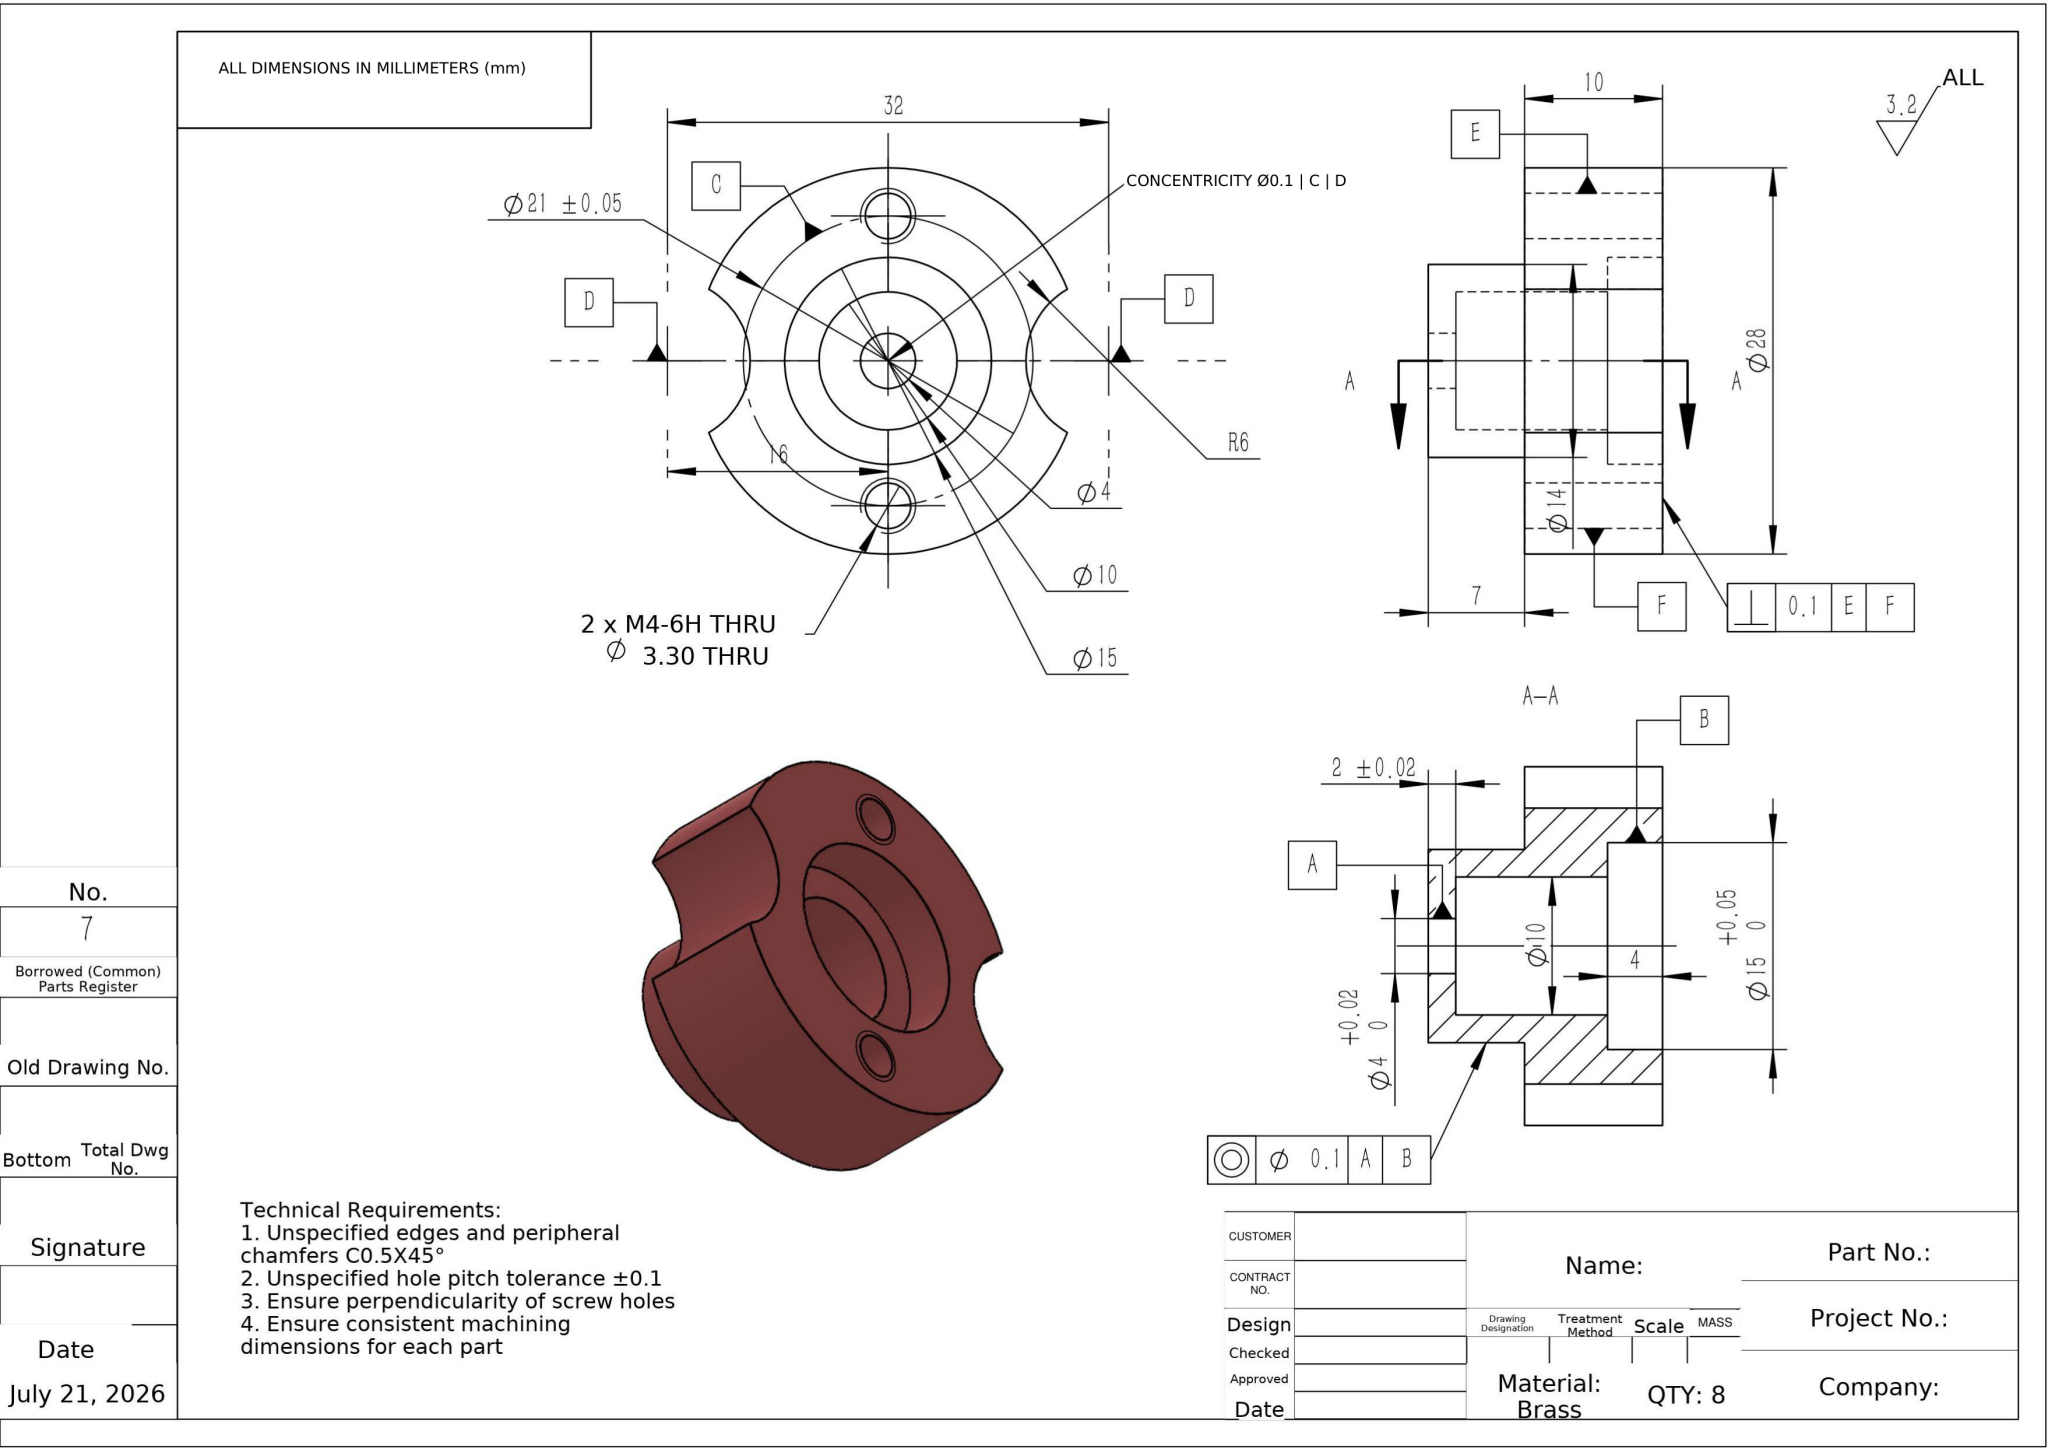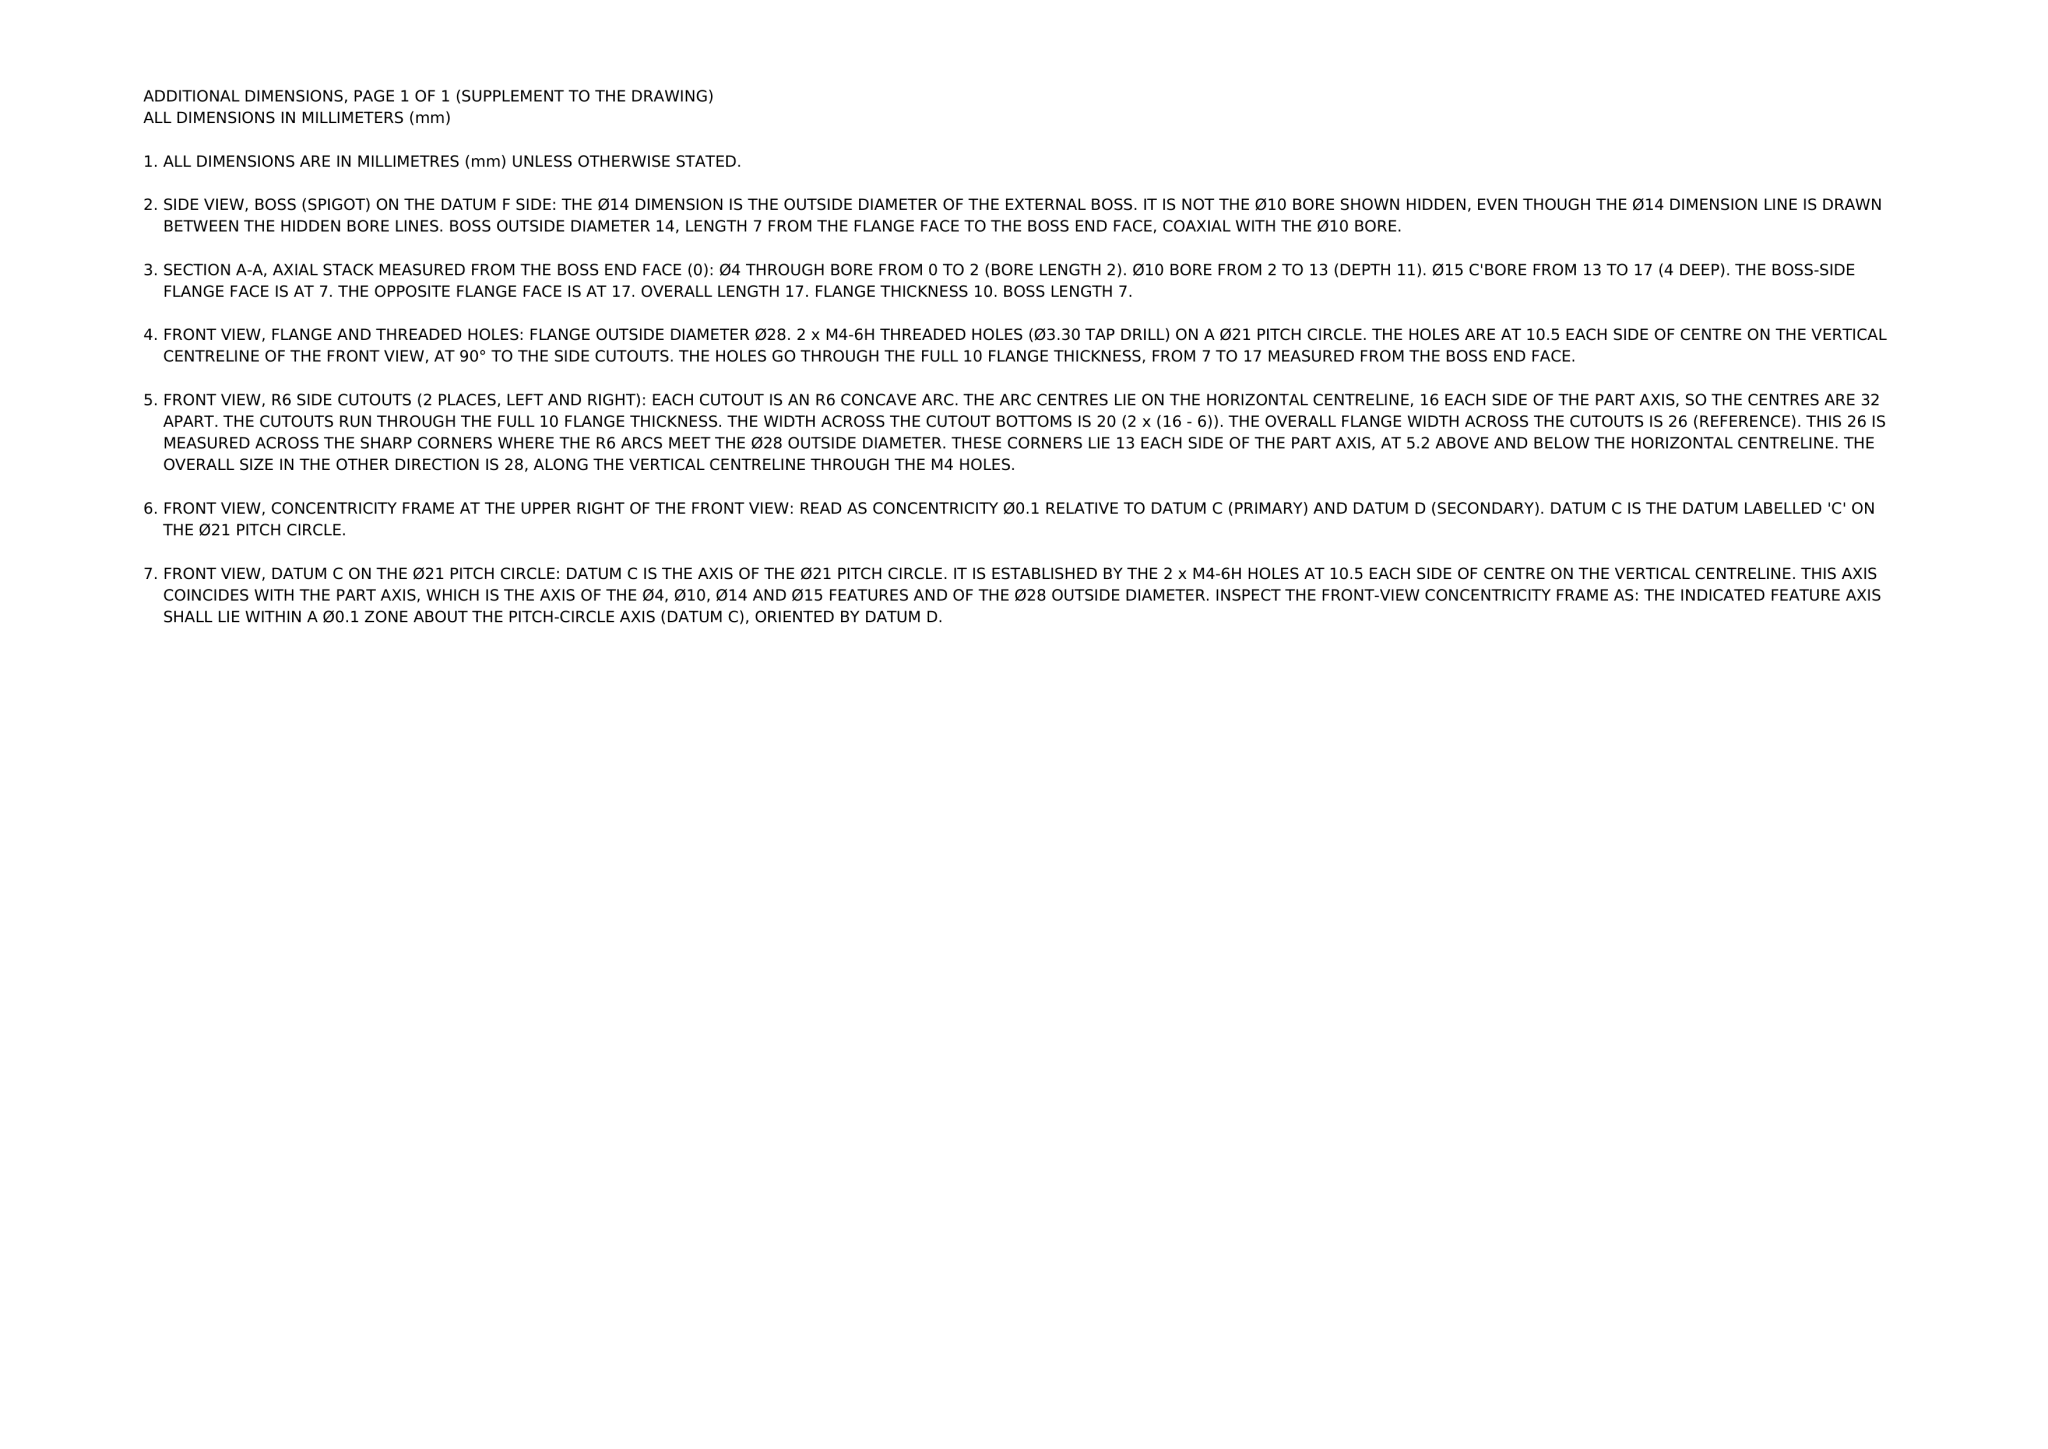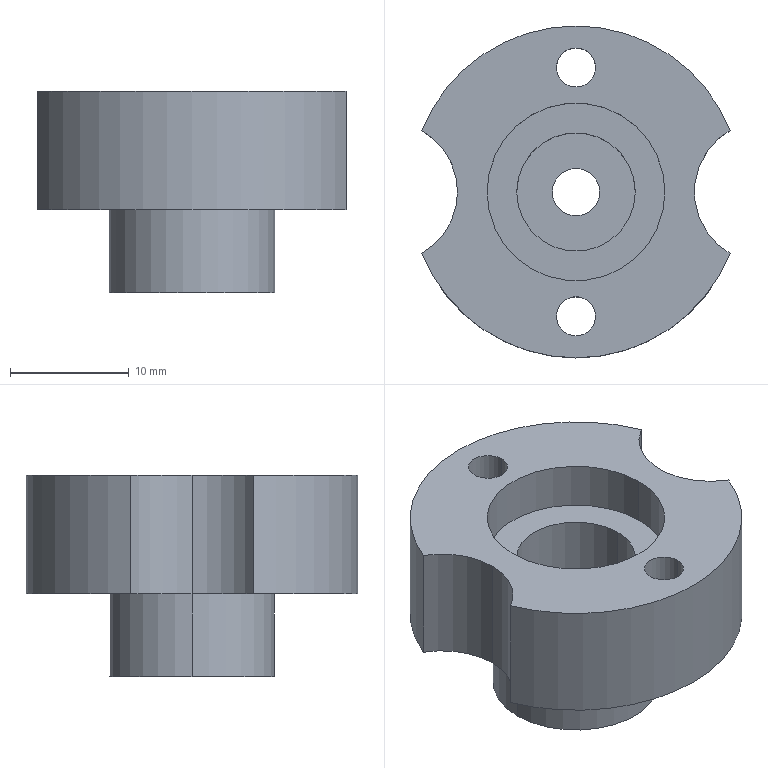Part | NX | mm | 1 solid | 22 faces | box 26 x 28 x 17 mm | volume 4886 mm3 | cylinder 17 | plane 5 | commonest cylinder face diameters 3.3 x4 12 x3 14 x2 4 x2 10 x2 15 x2 28 x2
STEP:
#1=CARTESIAN_POINT('',(1.65,10.5,7.));
#2=VERTEX_POINT('',#1);
#3=CARTESIAN_POINT('',(-1.65,10.5,7.));
#4=VERTEX_POINT('',#3);
#5=CARTESIAN_POINT('',(0.,10.5,7.));
#6=DIRECTION('',(0.,0.,-1.));
#7=DIRECTION('',(-1.,0.,0.));
#8=AXIS2_PLACEMENT_3D('',#5,#6,#7);
#9=CIRCLE('',#8,1.65);
#10=EDGE_CURVE('',#2,#4,#9,.T.);
#11=ORIENTED_EDGE('',*,*,#10,.T.);
#12=CARTESIAN_POINT('',(-1.65,10.5,17.));
#13=VERTEX_POINT('',#12);
#14=CARTESIAN_POINT('',(-1.65,10.5,17.));
#15=DIRECTION('',(0.,0.,1.));
#16=VECTOR('',#15,1000.);
#17=LINE('',#14,#16);
#18=EDGE_CURVE('',#4,#13,#17,.T.);
#19=ORIENTED_EDGE('',*,*,#18,.T.);
#20=CARTESIAN_POINT('',(1.65,10.5,17.));
#21=VERTEX_POINT('',#20);
#22=CARTESIAN_POINT('',(0.,10.5,17.));
#23=DIRECTION('',(0.,0.,1.));
#24=DIRECTION('',(1.,0.,0.));
#25=AXIS2_PLACEMENT_3D('',#22,#23,#24);
#26=CIRCLE('',#25,1.65);
#27=EDGE_CURVE('',#13,#21,#26,.T.);
#28=ORIENTED_EDGE('',*,*,#27,.T.);
#29=CARTESIAN_POINT('',(1.65,10.5,17.));
#30=DIRECTION('',(0.,0.,1.));
#31=VECTOR('',#30,1000.);
#32=LINE('',#29,#31);
#33=EDGE_CURVE('',#2,#21,#32,.T.);
#34=ORIENTED_EDGE('',*,*,#33,.F.);
#35=EDGE_LOOP('',(#11,#19,#28,#34));
#36=FACE_OUTER_BOUND('',#35,.T.);
#37=CARTESIAN_POINT('',(0.,10.5,17.));
#38=DIRECTION('',(0.,0.,1.));
#39=DIRECTION('',(1.,0.,0.));
#40=AXIS2_PLACEMENT_3D('',#37,#38,#39);
#41=CYLINDRICAL_SURFACE('',#40,1.65);
#42=ADVANCED_FACE('',(#36),#41,.F.);
#43=CARTESIAN_POINT('',(1.65,-10.5,7.));
#44=VERTEX_POINT('',#43);
#45=CARTESIAN_POINT('',(-1.65,-10.5,7.));
#46=VERTEX_POINT('',#45);
#47=CARTESIAN_POINT('',(0.,-10.5,7.));
#48=DIRECTION('',(0.,0.,-1.));
#49=DIRECTION('',(-1.,0.,0.));
#50=AXIS2_PLACEMENT_3D('',#47,#48,#49);
#51=CIRCLE('',#50,1.65);
#52=EDGE_CURVE('',#44,#46,#51,.T.);
#53=ORIENTED_EDGE('',*,*,#52,.T.);
#54=CARTESIAN_POINT('',(-1.65,-10.5,17.));
#55=VERTEX_POINT('',#54);
#56=CARTESIAN_POINT('',(-1.65,-10.5,17.));
#57=DIRECTION('',(0.,0.,1.));
#58=VECTOR('',#57,1000.);
#59=LINE('',#56,#58);
#60=EDGE_CURVE('',#46,#55,#59,.T.);
#61=ORIENTED_EDGE('',*,*,#60,.T.);
#62=CARTESIAN_POINT('',(1.65,-10.5,17.));
#63=VERTEX_POINT('',#62);
#64=CARTESIAN_POINT('',(0.,-10.5,17.));
#65=DIRECTION('',(0.,0.,1.));
#66=DIRECTION('',(1.,0.,0.));
#67=AXIS2_PLACEMENT_3D('',#64,#65,#66);
#68=CIRCLE('',#67,1.65);
#69=EDGE_CURVE('',#55,#63,#68,.T.);
#70=ORIENTED_EDGE('',*,*,#69,.T.);
#71=CARTESIAN_POINT('',(1.65,-10.5,17.));
#72=DIRECTION('',(0.,0.,1.));
#73=VECTOR('',#72,1000.);
#74=LINE('',#71,#73);
#75=EDGE_CURVE('',#44,#63,#74,.T.);
#76=ORIENTED_EDGE('',*,*,#75,.F.);
#77=EDGE_LOOP('',(#53,#61,#70,#76));
#78=FACE_OUTER_BOUND('',#77,.T.);
#79=CARTESIAN_POINT('',(0.,-10.5,17.));
#80=DIRECTION('',(0.,0.,1.));
#81=DIRECTION('',(1.,0.,0.));
#82=AXIS2_PLACEMENT_3D('',#79,#80,#81);
#83=CYLINDRICAL_SURFACE('',#82,1.65);
#84=ADVANCED_FACE('',(#78),#83,.F.);
#85=CARTESIAN_POINT('',(-7.,0.,7.));
#86=VERTEX_POINT('',#85);
#87=CARTESIAN_POINT('',(7.,0.,7.));
#88=VERTEX_POINT('',#87);
#89=CARTESIAN_POINT('',(0.,0.,7.));
#90=DIRECTION('',(0.,0.,-1.));
#91=DIRECTION('',(-1.,0.,0.));
#92=AXIS2_PLACEMENT_3D('',#89,#90,#91);
#93=CIRCLE('',#92,7.);
#94=EDGE_CURVE('',#86,#88,#93,.T.);
#95=ORIENTED_EDGE('',*,*,#94,.T.);
#96=CARTESIAN_POINT('',(7.,0.,0.));
#97=VERTEX_POINT('',#96);
#98=CARTESIAN_POINT('',(7.,0.,7.));
#99=DIRECTION('',(0.,0.,-1.));
#100=VECTOR('',#99,1000.);
#101=LINE('',#98,#100);
#102=EDGE_CURVE('',#88,#97,#101,.T.);
#103=ORIENTED_EDGE('',*,*,#102,.T.);
#104=CARTESIAN_POINT('',(-7.,0.,0.));
#105=VERTEX_POINT('',#104);
#106=CARTESIAN_POINT('',(0.,0.,0.));
#107=DIRECTION('',(0.,0.,-1.));
#108=DIRECTION('',(-1.,0.,0.));
#109=AXIS2_PLACEMENT_3D('',#106,#107,#108);
#110=CIRCLE('',#109,7.);
#111=EDGE_CURVE('',#105,#97,#110,.T.);
#112=ORIENTED_EDGE('',*,*,#111,.F.);
#113=CARTESIAN_POINT('',(-7.,0.,7.));
#114=DIRECTION('',(0.,0.,-1.));
#115=VECTOR('',#114,1000.);
#116=LINE('',#113,#115);
#117=EDGE_CURVE('',#86,#105,#116,.T.);
#118=ORIENTED_EDGE('',*,*,#117,.F.);
#119=EDGE_LOOP('',(#95,#103,#112,#118));
#120=FACE_OUTER_BOUND('',#119,.T.);
#121=CARTESIAN_POINT('',(0.,0.,7.));
#122=DIRECTION('',(0.,0.,-1.));
#123=DIRECTION('',(-1.,0.,0.));
#124=AXIS2_PLACEMENT_3D('',#121,#122,#123);
#125=CYLINDRICAL_SURFACE('',#124,7.);
#126=ADVANCED_FACE('',(#120),#125,.T.);
#127=CARTESIAN_POINT('',(-2.,0.,0.));
#128=VERTEX_POINT('',#127);
#129=CARTESIAN_POINT('',(2.,0.,0.));
#130=VERTEX_POINT('',#129);
#131=CARTESIAN_POINT('',(0.,0.,0.));
#132=DIRECTION('',(0.,0.,1.));
#133=DIRECTION('',(1.,0.,0.));
#134=AXIS2_PLACEMENT_3D('',#131,#132,#133);
#135=CIRCLE('',#134,2.);
#136=EDGE_CURVE('',#128,#130,#135,.T.);
#137=ORIENTED_EDGE('',*,*,#136,.F.);
#138=CARTESIAN_POINT('',(-2.,0.,2.));
#139=VERTEX_POINT('',#138);
#140=CARTESIAN_POINT('',(-2.,0.,0.));
#141=DIRECTION('',(0.,0.,1.));
#142=VECTOR('',#141,1000.);
#143=LINE('',#140,#142);
#144=EDGE_CURVE('',#128,#139,#143,.T.);
#145=ORIENTED_EDGE('',*,*,#144,.T.);
#146=CARTESIAN_POINT('',(2.,0.,2.));
#147=VERTEX_POINT('',#146);
#148=CARTESIAN_POINT('',(0.,0.,2.));
#149=DIRECTION('',(0.,0.,1.));
#150=DIRECTION('',(1.,0.,0.));
#151=AXIS2_PLACEMENT_3D('',#148,#149,#150);
#152=CIRCLE('',#151,2.);
#153=EDGE_CURVE('',#139,#147,#152,.T.);
#154=ORIENTED_EDGE('',*,*,#153,.T.);
#155=CARTESIAN_POINT('',(2.,0.,0.));
#156=DIRECTION('',(0.,0.,1.));
#157=VECTOR('',#156,1000.);
#158=LINE('',#155,#157);
#159=EDGE_CURVE('',#130,#147,#158,.T.);
#160=ORIENTED_EDGE('',*,*,#159,.F.);
#161=EDGE_LOOP('',(#137,#145,#154,#160));
#162=FACE_OUTER_BOUND('',#161,.T.);
#163=CARTESIAN_POINT('',(0.,0.,0.));
#164=DIRECTION('',(0.,0.,1.));
#165=DIRECTION('',(1.,0.,0.));
#166=AXIS2_PLACEMENT_3D('',#163,#164,#165);
#167=CYLINDRICAL_SURFACE('',#166,2.);
#168=ADVANCED_FACE('',(#162),#167,.F.);
#169=CARTESIAN_POINT('',(-5.,0.,2.));
#170=VERTEX_POINT('',#169);
#171=CARTESIAN_POINT('',(5.,0.,2.));
#172=VERTEX_POINT('',#171);
#173=CARTESIAN_POINT('',(0.,0.,2.));
#174=DIRECTION('',(0.,0.,1.));
#175=DIRECTION('',(1.,0.,0.));
#176=AXIS2_PLACEMENT_3D('',#173,#174,#175);
#177=CIRCLE('',#176,5.);
#178=EDGE_CURVE('',#170,#172,#177,.T.);
#179=ORIENTED_EDGE('',*,*,#178,.F.);
#180=CARTESIAN_POINT('',(-5.,0.,13.));
#181=VERTEX_POINT('',#180);
#182=CARTESIAN_POINT('',(-5.,0.,2.));
#183=DIRECTION('',(0.,0.,1.));
#184=VECTOR('',#183,1000.);
#185=LINE('',#182,#184);
#186=EDGE_CURVE('',#170,#181,#185,.T.);
#187=ORIENTED_EDGE('',*,*,#186,.T.);
#188=CARTESIAN_POINT('',(5.,0.,13.));
#189=VERTEX_POINT('',#188);
#190=CARTESIAN_POINT('',(0.,0.,13.));
#191=DIRECTION('',(0.,0.,1.));
#192=DIRECTION('',(1.,0.,0.));
#193=AXIS2_PLACEMENT_3D('',#190,#191,#192);
#194=CIRCLE('',#193,5.);
#195=EDGE_CURVE('',#181,#189,#194,.T.);
#196=ORIENTED_EDGE('',*,*,#195,.T.);
#197=CARTESIAN_POINT('',(5.,0.,2.));
#198=DIRECTION('',(0.,0.,1.));
#199=VECTOR('',#198,1000.);
#200=LINE('',#197,#199);
#201=EDGE_CURVE('',#172,#189,#200,.T.);
#202=ORIENTED_EDGE('',*,*,#201,.F.);
#203=EDGE_LOOP('',(#179,#187,#196,#202));
#204=FACE_OUTER_BOUND('',#203,.T.);
#205=CARTESIAN_POINT('',(0.,0.,2.));
#206=DIRECTION('',(0.,0.,1.));
#207=DIRECTION('',(1.,0.,0.));
#208=AXIS2_PLACEMENT_3D('',#205,#206,#207);
#209=CYLINDRICAL_SURFACE('',#208,5.);
#210=ADVANCED_FACE('',(#204),#209,.F.);
#211=CARTESIAN_POINT('',(-7.5,0.,13.));
#212=VERTEX_POINT('',#211);
#213=CARTESIAN_POINT('',(7.5,0.,13.));
#214=VERTEX_POINT('',#213);
#215=CARTESIAN_POINT('',(0.,0.,13.));
#216=DIRECTION('',(0.,0.,1.));
#217=DIRECTION('',(1.,0.,0.));
#218=AXIS2_PLACEMENT_3D('',#215,#216,#217);
#219=CIRCLE('',#218,7.5);
#220=EDGE_CURVE('',#212,#214,#219,.T.);
#221=ORIENTED_EDGE('',*,*,#220,.F.);
#222=CARTESIAN_POINT('',(-7.5,0.,17.));
#223=VERTEX_POINT('',#222);
#224=CARTESIAN_POINT('',(-7.5,0.,13.));
#225=DIRECTION('',(0.,0.,1.));
#226=VECTOR('',#225,1000.);
#227=LINE('',#224,#226);
#228=EDGE_CURVE('',#212,#223,#227,.T.);
#229=ORIENTED_EDGE('',*,*,#228,.T.);
#230=CARTESIAN_POINT('',(7.5,0.,17.));
#231=VERTEX_POINT('',#230);
#232=CARTESIAN_POINT('',(0.,0.,17.));
#233=DIRECTION('',(0.,0.,1.));
#234=DIRECTION('',(1.,0.,0.));
#235=AXIS2_PLACEMENT_3D('',#232,#233,#234);
#236=CIRCLE('',#235,7.5);
#237=EDGE_CURVE('',#223,#231,#236,.T.);
#238=ORIENTED_EDGE('',*,*,#237,.T.);
#239=CARTESIAN_POINT('',(7.5,0.,13.));
#240=DIRECTION('',(0.,0.,1.));
#241=VECTOR('',#240,1000.);
#242=LINE('',#239,#241);
#243=EDGE_CURVE('',#214,#231,#242,.T.);
#244=ORIENTED_EDGE('',*,*,#243,.F.);
#245=EDGE_LOOP('',(#221,#229,#238,#244));
#246=FACE_OUTER_BOUND('',#245,.T.);
#247=CARTESIAN_POINT('',(0.,0.,13.));
#248=DIRECTION('',(0.,0.,1.));
#249=DIRECTION('',(1.,0.,0.));
#250=AXIS2_PLACEMENT_3D('',#247,#248,#249);
#251=CYLINDRICAL_SURFACE('',#250,7.5);
#252=ADVANCED_FACE('',(#246),#251,.F.);
#253=CARTESIAN_POINT('',(-10.,0.,7.));
#254=VERTEX_POINT('',#253);
#255=CARTESIAN_POINT('',(-13.,5.196,7.));
#256=VERTEX_POINT('',#255);
#257=CARTESIAN_POINT('',(-16.,0.,7.));
#258=DIRECTION('',(0.,0.,1.));
#259=DIRECTION('',(-1.,0.,0.));
#260=AXIS2_PLACEMENT_3D('',#257,#258,#259);
#261=CIRCLE('',#260,6.);
#262=EDGE_CURVE('',#254,#256,#261,.T.);
#263=ORIENTED_EDGE('',*,*,#262,.F.);
#264=CARTESIAN_POINT('',(-10.,0.,17.));
#265=VERTEX_POINT('',#264);
#266=CARTESIAN_POINT('',(-10.,0.,0.));
#267=DIRECTION('',(0.,0.,1.));
#268=VECTOR('',#267,1000.);
#269=LINE('',#266,#268);
#270=EDGE_CURVE('',#254,#265,#269,.T.);
#271=ORIENTED_EDGE('',*,*,#270,.T.);
#272=CARTESIAN_POINT('',(-13.,5.196,17.));
#273=VERTEX_POINT('',#272);
#274=CARTESIAN_POINT('',(-16.,0.,17.));
#275=DIRECTION('',(0.,0.,1.));
#276=DIRECTION('',(1.,0.,0.));
#277=AXIS2_PLACEMENT_3D('',#274,#275,#276);
#278=CIRCLE('',#277,6.);
#279=EDGE_CURVE('',#265,#273,#278,.T.);
#280=ORIENTED_EDGE('',*,*,#279,.T.);
#281=CARTESIAN_POINT('',(-13.,5.196,8.5));
#282=DIRECTION('',(0.,0.,1.));
#283=VECTOR('',#282,1000.);
#284=LINE('',#281,#283);
#285=EDGE_CURVE('',#256,#273,#284,.T.);
#286=ORIENTED_EDGE('',*,*,#285,.F.);
#287=EDGE_LOOP('',(#263,#271,#280,#286));
#288=FACE_OUTER_BOUND('',#287,.T.);
#289=CARTESIAN_POINT('',(-16.,0.,0.));
#290=DIRECTION('',(0.,0.,1.));
#291=DIRECTION('',(1.,0.,0.));
#292=AXIS2_PLACEMENT_3D('',#289,#290,#291);
#293=CYLINDRICAL_SURFACE('',#292,6.);
#294=ADVANCED_FACE('',(#288),#293,.F.);
#295=CARTESIAN_POINT('',(13.,-5.196,7.));
#296=VERTEX_POINT('',#295);
#297=CARTESIAN_POINT('',(-13.,-5.196,7.));
#298=VERTEX_POINT('',#297);
#299=CARTESIAN_POINT('',(0.,0.,7.));
#300=DIRECTION('',(0.,0.,-1.));
#301=DIRECTION('',(-1.,0.,0.));
#302=AXIS2_PLACEMENT_3D('',#299,#300,#301);
#303=CIRCLE('',#302,14.);
#304=EDGE_CURVE('',#296,#298,#303,.T.);
#305=ORIENTED_EDGE('',*,*,#304,.F.);
#306=CARTESIAN_POINT('',(13.,-5.196,17.));
#307=VERTEX_POINT('',#306);
#308=CARTESIAN_POINT('',(13.,-5.196,8.5));
#309=DIRECTION('',(0.,0.,1.));
#310=VECTOR('',#309,1000.);
#311=LINE('',#308,#310);
#312=EDGE_CURVE('',#296,#307,#311,.T.);
#313=ORIENTED_EDGE('',*,*,#312,.T.);
#314=CARTESIAN_POINT('',(-13.,-5.196,17.));
#315=VERTEX_POINT('',#314);
#316=CARTESIAN_POINT('',(0.,0.,17.));
#317=DIRECTION('',(0.,0.,1.));
#318=DIRECTION('',(1.,0.,0.));
#319=AXIS2_PLACEMENT_3D('',#316,#317,#318);
#320=CIRCLE('',#319,14.);
#321=EDGE_CURVE('',#315,#307,#320,.T.);
#322=ORIENTED_EDGE('',*,*,#321,.F.);
#323=CARTESIAN_POINT('',(-13.,-5.196,8.5));
#324=DIRECTION('',(0.,0.,-1.));
#325=VECTOR('',#324,1000.);
#326=LINE('',#323,#325);
#327=EDGE_CURVE('',#315,#298,#326,.T.);
#328=ORIENTED_EDGE('',*,*,#327,.T.);
#329=EDGE_LOOP('',(#305,#313,#322,#328));
#330=FACE_OUTER_BOUND('',#329,.T.);
#331=CARTESIAN_POINT('',(0.,0.,17.));
#332=DIRECTION('',(0.,0.,-1.));
#333=DIRECTION('',(-1.,0.,0.));
#334=AXIS2_PLACEMENT_3D('',#331,#332,#333);
#335=CYLINDRICAL_SURFACE('',#334,14.);
#336=ADVANCED_FACE('',(#330),#335,.T.);
#337=CARTESIAN_POINT('',(13.,5.196,7.));
#338=VERTEX_POINT('',#337);
#339=CARTESIAN_POINT('',(0.,0.,7.));
#340=DIRECTION('',(0.,0.,-1.));
#341=DIRECTION('',(-1.,0.,0.));
#342=AXIS2_PLACEMENT_3D('',#339,#340,#341);
#343=CIRCLE('',#342,14.);
#344=EDGE_CURVE('',#256,#338,#343,.T.);
#345=ORIENTED_EDGE('',*,*,#344,.F.);
#346=ORIENTED_EDGE('',*,*,#285,.T.);
#347=CARTESIAN_POINT('',(13.,5.196,17.));
#348=VERTEX_POINT('',#347);
#349=CARTESIAN_POINT('',(0.,0.,17.));
#350=DIRECTION('',(0.,0.,1.));
#351=DIRECTION('',(1.,0.,0.));
#352=AXIS2_PLACEMENT_3D('',#349,#350,#351);
#353=CIRCLE('',#352,14.);
#354=EDGE_CURVE('',#348,#273,#353,.T.);
#355=ORIENTED_EDGE('',*,*,#354,.F.);
#356=CARTESIAN_POINT('',(13.,5.196,8.5));
#357=DIRECTION('',(0.,0.,-1.));
#358=VECTOR('',#357,1000.);
#359=LINE('',#356,#358);
#360=EDGE_CURVE('',#348,#338,#359,.T.);
#361=ORIENTED_EDGE('',*,*,#360,.T.);
#362=EDGE_LOOP('',(#345,#346,#355,#361));
#363=FACE_OUTER_BOUND('',#362,.T.);
#364=CARTESIAN_POINT('',(0.,0.,17.));
#365=DIRECTION('',(0.,0.,-1.));
#366=DIRECTION('',(-1.,0.,0.));
#367=AXIS2_PLACEMENT_3D('',#364,#365,#366);
#368=CYLINDRICAL_SURFACE('',#367,14.);
#369=ADVANCED_FACE('',(#363),#368,.T.);
#370=CARTESIAN_POINT('',(0.,0.,0.));
#371=DIRECTION('',(0.,0.,1.));
#372=DIRECTION('',(1.,0.,0.));
#373=AXIS2_PLACEMENT_3D('',#370,#371,#372);
#374=CIRCLE('',#373,2.);
#375=EDGE_CURVE('',#130,#128,#374,.T.);
#376=ORIENTED_EDGE('',*,*,#375,.T.);
#377=ORIENTED_EDGE('',*,*,#136,.T.);
#378=EDGE_LOOP('',(#376,#377));
#379=FACE_BOUND('',#378,.T.);
#380=ORIENTED_EDGE('',*,*,#111,.T.);
#381=CARTESIAN_POINT('',(0.,0.,0.));
#382=DIRECTION('',(0.,0.,-1.));
#383=DIRECTION('',(-1.,0.,0.));
#384=AXIS2_PLACEMENT_3D('',#381,#382,#383);
#385=CIRCLE('',#384,7.);
#386=EDGE_CURVE('',#97,#105,#385,.T.);
#387=ORIENTED_EDGE('',*,*,#386,.T.);
#388=EDGE_LOOP('',(#380,#387));
#389=FACE_OUTER_BOUND('',#388,.T.);
#390=CARTESIAN_POINT('',(0.,0.,0.));
#391=DIRECTION('',(0.,0.,1.));
#392=DIRECTION('',(1.,0.,0.));
#393=AXIS2_PLACEMENT_3D('',#390,#391,#392);
#394=PLANE('',#393);
#395=ADVANCED_FACE('',(#379,#389),#394,.F.);
#396=ORIENTED_EDGE('',*,*,#270,.F.);
#397=CARTESIAN_POINT('',(-16.,0.,7.));
#398=DIRECTION('',(0.,0.,1.));
#399=DIRECTION('',(-1.,0.,0.));
#400=AXIS2_PLACEMENT_3D('',#397,#398,#399);
#401=CIRCLE('',#400,6.);
#402=EDGE_CURVE('',#298,#254,#401,.T.);
#403=ORIENTED_EDGE('',*,*,#402,.F.);
#404=ORIENTED_EDGE('',*,*,#327,.F.);
#405=CARTESIAN_POINT('',(-16.,0.,17.));
#406=DIRECTION('',(0.,0.,1.));
#407=DIRECTION('',(1.,0.,0.));
#408=AXIS2_PLACEMENT_3D('',#405,#406,#407);
#409=CIRCLE('',#408,6.);
#410=EDGE_CURVE('',#315,#265,#409,.T.);
#411=ORIENTED_EDGE('',*,*,#410,.T.);
#412=EDGE_LOOP('',(#396,#403,#404,#411));
#413=FACE_OUTER_BOUND('',#412,.T.);
#414=CARTESIAN_POINT('',(-16.,0.,0.));
#415=DIRECTION('',(0.,0.,1.));
#416=DIRECTION('',(1.,0.,0.));
#417=AXIS2_PLACEMENT_3D('',#414,#415,#416);
#418=CYLINDRICAL_SURFACE('',#417,6.);
#419=ADVANCED_FACE('',(#413),#418,.F.);
#420=CARTESIAN_POINT('',(16.,0.,7.));
#421=DIRECTION('',(0.,0.,1.));
#422=DIRECTION('',(-1.,0.,0.));
#423=AXIS2_PLACEMENT_3D('',#420,#421,#422);
#424=CIRCLE('',#423,6.);
#425=EDGE_CURVE('',#338,#296,#424,.T.);
#426=ORIENTED_EDGE('',*,*,#425,.F.);
#427=ORIENTED_EDGE('',*,*,#360,.F.);
#428=CARTESIAN_POINT('',(16.,0.,17.));
#429=DIRECTION('',(0.,0.,1.));
#430=DIRECTION('',(1.,0.,0.));
#431=AXIS2_PLACEMENT_3D('',#428,#429,#430);
#432=CIRCLE('',#431,6.);
#433=EDGE_CURVE('',#348,#307,#432,.T.);
#434=ORIENTED_EDGE('',*,*,#433,.T.);
#435=ORIENTED_EDGE('',*,*,#312,.F.);
#436=EDGE_LOOP('',(#426,#427,#434,#435));
#437=FACE_OUTER_BOUND('',#436,.T.);
#438=CARTESIAN_POINT('',(16.,0.,0.));
#439=DIRECTION('',(0.,0.,1.));
#440=DIRECTION('',(1.,0.,0.));
#441=AXIS2_PLACEMENT_3D('',#438,#439,#440);
#442=CYLINDRICAL_SURFACE('',#441,6.);
#443=ADVANCED_FACE('',(#437),#442,.F.);
#444=CARTESIAN_POINT('',(0.,10.5,17.));
#445=DIRECTION('',(0.,0.,1.));
#446=DIRECTION('',(1.,0.,0.));
#447=AXIS2_PLACEMENT_3D('',#444,#445,#446);
#448=CIRCLE('',#447,1.65);
#449=EDGE_CURVE('',#21,#13,#448,.T.);
#450=ORIENTED_EDGE('',*,*,#449,.F.);
#451=ORIENTED_EDGE('',*,*,#27,.F.);
#452=EDGE_LOOP('',(#450,#451));
#453=FACE_BOUND('',#452,.T.);
#454=CARTESIAN_POINT('',(0.,-10.5,17.));
#455=DIRECTION('',(0.,0.,1.));
#456=DIRECTION('',(1.,0.,0.));
#457=AXIS2_PLACEMENT_3D('',#454,#455,#456);
#458=CIRCLE('',#457,1.65);
#459=EDGE_CURVE('',#63,#55,#458,.T.);
#460=ORIENTED_EDGE('',*,*,#459,.F.);
#461=ORIENTED_EDGE('',*,*,#69,.F.);
#462=EDGE_LOOP('',(#460,#461));
#463=FACE_BOUND('',#462,.T.);
#464=ORIENTED_EDGE('',*,*,#433,.F.);
#465=ORIENTED_EDGE('',*,*,#354,.T.);
#466=ORIENTED_EDGE('',*,*,#279,.F.);
#467=ORIENTED_EDGE('',*,*,#410,.F.);
#468=ORIENTED_EDGE('',*,*,#321,.T.);
#469=EDGE_LOOP('',(#464,#465,#466,#467,#468));
#470=FACE_OUTER_BOUND('',#469,.T.);
#471=CARTESIAN_POINT('',(0.,0.,17.));
#472=DIRECTION('',(0.,0.,1.));
#473=DIRECTION('',(1.,0.,0.));
#474=AXIS2_PLACEMENT_3D('',#471,#472,#473);
#475=CIRCLE('',#474,7.5);
#476=EDGE_CURVE('',#231,#223,#475,.T.);
#477=ORIENTED_EDGE('',*,*,#476,.F.);
#478=ORIENTED_EDGE('',*,*,#237,.F.);
#479=EDGE_LOOP('',(#477,#478));
#480=FACE_BOUND('',#479,.T.);
#481=CARTESIAN_POINT('',(0.,0.,17.));
#482=DIRECTION('',(0.,0.,1.));
#483=DIRECTION('',(1.,0.,0.));
#484=AXIS2_PLACEMENT_3D('',#481,#482,#483);
#485=PLANE('',#484);
#486=ADVANCED_FACE('',(#453,#463,#470,#480),#485,.T.);
#487=ORIENTED_EDGE('',*,*,#228,.F.);
#488=CARTESIAN_POINT('',(0.,0.,13.));
#489=DIRECTION('',(0.,0.,1.));
#490=DIRECTION('',(1.,0.,0.));
#491=AXIS2_PLACEMENT_3D('',#488,#489,#490);
#492=CIRCLE('',#491,7.5);
#493=EDGE_CURVE('',#214,#212,#492,.T.);
#494=ORIENTED_EDGE('',*,*,#493,.F.);
#495=ORIENTED_EDGE('',*,*,#243,.T.);
#496=ORIENTED_EDGE('',*,*,#476,.T.);
#497=EDGE_LOOP('',(#487,#494,#495,#496));
#498=FACE_OUTER_BOUND('',#497,.T.);
#499=CARTESIAN_POINT('',(0.,0.,13.));
#500=DIRECTION('',(0.,0.,1.));
#501=DIRECTION('',(1.,0.,0.));
#502=AXIS2_PLACEMENT_3D('',#499,#500,#501);
#503=CYLINDRICAL_SURFACE('',#502,7.5);
#504=ADVANCED_FACE('',(#498),#503,.F.);
#505=CARTESIAN_POINT('',(0.,0.,13.));
#506=DIRECTION('',(0.,0.,1.));
#507=DIRECTION('',(1.,0.,0.));
#508=AXIS2_PLACEMENT_3D('',#505,#506,#507);
#509=CIRCLE('',#508,5.);
#510=EDGE_CURVE('',#189,#181,#509,.T.);
#511=ORIENTED_EDGE('',*,*,#510,.F.);
#512=ORIENTED_EDGE('',*,*,#195,.F.);
#513=EDGE_LOOP('',(#511,#512));
#514=FACE_BOUND('',#513,.T.);
#515=ORIENTED_EDGE('',*,*,#493,.T.);
#516=ORIENTED_EDGE('',*,*,#220,.T.);
#517=EDGE_LOOP('',(#515,#516));
#518=FACE_OUTER_BOUND('',#517,.T.);
#519=CARTESIAN_POINT('',(0.,0.,13.));
#520=DIRECTION('',(0.,0.,1.));
#521=DIRECTION('',(1.,0.,0.));
#522=AXIS2_PLACEMENT_3D('',#519,#520,#521);
#523=PLANE('',#522);
#524=ADVANCED_FACE('',(#514,#518),#523,.T.);
#525=ORIENTED_EDGE('',*,*,#186,.F.);
#526=CARTESIAN_POINT('',(0.,0.,2.));
#527=DIRECTION('',(0.,0.,1.));
#528=DIRECTION('',(1.,0.,0.));
#529=AXIS2_PLACEMENT_3D('',#526,#527,#528);
#530=CIRCLE('',#529,5.);
#531=EDGE_CURVE('',#172,#170,#530,.T.);
#532=ORIENTED_EDGE('',*,*,#531,.F.);
#533=ORIENTED_EDGE('',*,*,#201,.T.);
#534=ORIENTED_EDGE('',*,*,#510,.T.);
#535=EDGE_LOOP('',(#525,#532,#533,#534));
#536=FACE_OUTER_BOUND('',#535,.T.);
#537=CARTESIAN_POINT('',(0.,0.,2.));
#538=DIRECTION('',(0.,0.,1.));
#539=DIRECTION('',(1.,0.,0.));
#540=AXIS2_PLACEMENT_3D('',#537,#538,#539);
#541=CYLINDRICAL_SURFACE('',#540,5.);
#542=ADVANCED_FACE('',(#536),#541,.F.);
#543=CARTESIAN_POINT('',(0.,0.,2.));
#544=DIRECTION('',(0.,0.,1.));
#545=DIRECTION('',(1.,0.,0.));
#546=AXIS2_PLACEMENT_3D('',#543,#544,#545);
#547=CIRCLE('',#546,2.);
#548=EDGE_CURVE('',#147,#139,#547,.T.);
#549=ORIENTED_EDGE('',*,*,#548,.F.);
#550=ORIENTED_EDGE('',*,*,#153,.F.);
#551=EDGE_LOOP('',(#549,#550));
#552=FACE_BOUND('',#551,.T.);
#553=ORIENTED_EDGE('',*,*,#531,.T.);
#554=ORIENTED_EDGE('',*,*,#178,.T.);
#555=EDGE_LOOP('',(#553,#554));
#556=FACE_OUTER_BOUND('',#555,.T.);
#557=CARTESIAN_POINT('',(0.,0.,2.));
#558=DIRECTION('',(0.,0.,1.));
#559=DIRECTION('',(1.,0.,0.));
#560=AXIS2_PLACEMENT_3D('',#557,#558,#559);
#561=PLANE('',#560);
#562=ADVANCED_FACE('',(#552,#556),#561,.T.);
#563=ORIENTED_EDGE('',*,*,#144,.F.);
#564=ORIENTED_EDGE('',*,*,#375,.F.);
#565=ORIENTED_EDGE('',*,*,#159,.T.);
#566=ORIENTED_EDGE('',*,*,#548,.T.);
#567=EDGE_LOOP('',(#563,#564,#565,#566));
#568=FACE_OUTER_BOUND('',#567,.T.);
#569=CARTESIAN_POINT('',(0.,0.,0.));
#570=DIRECTION('',(0.,0.,1.));
#571=DIRECTION('',(1.,0.,0.));
#572=AXIS2_PLACEMENT_3D('',#569,#570,#571);
#573=CYLINDRICAL_SURFACE('',#572,2.);
#574=ADVANCED_FACE('',(#568),#573,.F.);
#575=ORIENTED_EDGE('',*,*,#10,.F.);
#576=CARTESIAN_POINT('',(0.,10.5,7.));
#577=DIRECTION('',(0.,0.,-1.));
#578=DIRECTION('',(-1.,0.,0.));
#579=AXIS2_PLACEMENT_3D('',#576,#577,#578);
#580=CIRCLE('',#579,1.65);
#581=EDGE_CURVE('',#4,#2,#580,.T.);
#582=ORIENTED_EDGE('',*,*,#581,.F.);
#583=EDGE_LOOP('',(#575,#582));
#584=FACE_BOUND('',#583,.T.);
#585=ORIENTED_EDGE('',*,*,#52,.F.);
#586=CARTESIAN_POINT('',(0.,-10.5,7.));
#587=DIRECTION('',(0.,0.,-1.));
#588=DIRECTION('',(-1.,0.,0.));
#589=AXIS2_PLACEMENT_3D('',#586,#587,#588);
#590=CIRCLE('',#589,1.65);
#591=EDGE_CURVE('',#46,#44,#590,.T.);
#592=ORIENTED_EDGE('',*,*,#591,.F.);
#593=EDGE_LOOP('',(#585,#592));
#594=FACE_BOUND('',#593,.T.);
#595=ORIENTED_EDGE('',*,*,#94,.F.);
#596=CARTESIAN_POINT('',(0.,0.,7.));
#597=DIRECTION('',(0.,0.,-1.));
#598=DIRECTION('',(-1.,0.,0.));
#599=AXIS2_PLACEMENT_3D('',#596,#597,#598);
#600=CIRCLE('',#599,7.);
#601=EDGE_CURVE('',#88,#86,#600,.T.);
#602=ORIENTED_EDGE('',*,*,#601,.F.);
#603=EDGE_LOOP('',(#595,#602));
#604=FACE_BOUND('',#603,.T.);
#605=ORIENTED_EDGE('',*,*,#402,.T.);
#606=ORIENTED_EDGE('',*,*,#262,.T.);
#607=ORIENTED_EDGE('',*,*,#344,.T.);
#608=ORIENTED_EDGE('',*,*,#425,.T.);
#609=ORIENTED_EDGE('',*,*,#304,.T.);
#610=EDGE_LOOP('',(#605,#606,#607,#608,#609));
#611=FACE_OUTER_BOUND('',#610,.T.);
#612=CARTESIAN_POINT('',(-8.,0.,7.));
#613=DIRECTION('',(0.,0.,-1.));
#614=DIRECTION('',(-1.,0.,0.));
#615=AXIS2_PLACEMENT_3D('',#612,#613,#614);
#616=PLANE('',#615);
#617=ADVANCED_FACE('',(#584,#594,#604,#611),#616,.T.);
#618=ORIENTED_EDGE('',*,*,#102,.F.);
#619=ORIENTED_EDGE('',*,*,#601,.T.);
#620=ORIENTED_EDGE('',*,*,#117,.T.);
#621=ORIENTED_EDGE('',*,*,#386,.F.);
#622=EDGE_LOOP('',(#618,#619,#620,#621));
#623=FACE_OUTER_BOUND('',#622,.T.);
#624=CARTESIAN_POINT('',(0.,0.,7.));
#625=DIRECTION('',(0.,0.,-1.));
#626=DIRECTION('',(-1.,0.,0.));
#627=AXIS2_PLACEMENT_3D('',#624,#625,#626);
#628=CYLINDRICAL_SURFACE('',#627,7.);
#629=ADVANCED_FACE('',(#623),#628,.T.);
#630=ORIENTED_EDGE('',*,*,#60,.F.);
#631=ORIENTED_EDGE('',*,*,#591,.T.);
#632=ORIENTED_EDGE('',*,*,#75,.T.);
#633=ORIENTED_EDGE('',*,*,#459,.T.);
#634=EDGE_LOOP('',(#630,#631,#632,#633));
#635=FACE_OUTER_BOUND('',#634,.T.);
#636=CARTESIAN_POINT('',(0.,-10.5,17.));
#637=DIRECTION('',(0.,0.,1.));
#638=DIRECTION('',(1.,0.,0.));
#639=AXIS2_PLACEMENT_3D('',#636,#637,#638);
#640=CYLINDRICAL_SURFACE('',#639,1.65);
#641=ADVANCED_FACE('',(#635),#640,.F.);
#642=ORIENTED_EDGE('',*,*,#18,.F.);
#643=ORIENTED_EDGE('',*,*,#581,.T.);
#644=ORIENTED_EDGE('',*,*,#33,.T.);
#645=ORIENTED_EDGE('',*,*,#449,.T.);
#646=EDGE_LOOP('',(#642,#643,#644,#645));
#647=FACE_OUTER_BOUND('',#646,.T.);
#648=CARTESIAN_POINT('',(0.,10.5,17.));
#649=DIRECTION('',(0.,0.,1.));
#650=DIRECTION('',(1.,0.,0.));
#651=AXIS2_PLACEMENT_3D('',#648,#649,#650);
#652=CYLINDRICAL_SURFACE('',#651,1.65);
#653=ADVANCED_FACE('',(#647),#652,.F.);
#654=CLOSED_SHELL('',(#42,#84,#126,#168,#210,#252,#294,#336,#369,#395,#419,#443,#486,#504,#524,#542,#562,#574,#617,#629,#641,#653));
#655=MANIFOLD_SOLID_BREP('',#654);
#656=CARTESIAN_POINT('',(0.,0.,0.));
#657=DIRECTION('',(0.,0.,1.));
#658=DIRECTION('',(1.,0.,0.));
#659=AXIS2_PLACEMENT_3D('',#656,#657,#658);
#660=(LENGTH_UNIT()NAMED_UNIT(*)SI_UNIT(.MILLI.,.METRE.));
#661=UNCERTAINTY_MEASURE_WITH_UNIT(LENGTH_MEASURE(0.00001),#660,'','');
#662=(NAMED_UNIT(*)PLANE_ANGLE_UNIT()SI_UNIT($,.RADIAN.));
#663=(NAMED_UNIT(*)SI_UNIT($,.STERADIAN.)SOLID_ANGLE_UNIT());
#664=(GEOMETRIC_REPRESENTATION_CONTEXT(3)GLOBAL_UNCERTAINTY_ASSIGNED_CONTEXT((#661))GLOBAL_UNIT_ASSIGNED_CONTEXT((#660,#662,#663))REPRESENTATION_CONTEXT('',''));
#665=ADVANCED_BREP_SHAPE_REPRESENTATION('',(#655,#659),#664);
#666=COLOUR_RGB('',0.7922,0.8196,0.9333);
#667=FILL_AREA_STYLE_COLOUR('',#666);
#668=FILL_AREA_STYLE('',(#667));
#669=SURFACE_STYLE_FILL_AREA(#668);
#670=SURFACE_SIDE_STYLE('',(#669));
#671=SURFACE_STYLE_USAGE(.BOTH.,#670);
#672=PRESENTATION_STYLE_ASSIGNMENT((#671));
#673=STYLED_ITEM('',(#672),#655);
#674=(LENGTH_UNIT()NAMED_UNIT(*)SI_UNIT(.MILLI.,.METRE.));
#675=UNCERTAINTY_MEASURE_WITH_UNIT(LENGTH_MEASURE(0.00001),#674,'','');
#676=(NAMED_UNIT(*)PLANE_ANGLE_UNIT()SI_UNIT($,.RADIAN.));
#677=(NAMED_UNIT(*)SI_UNIT($,.STERADIAN.)SOLID_ANGLE_UNIT());
#678=(GEOMETRIC_REPRESENTATION_CONTEXT(3)GLOBAL_UNCERTAINTY_ASSIGNED_CONTEXT((#675))GLOBAL_UNIT_ASSIGNED_CONTEXT((#674,#676,#677))REPRESENTATION_CONTEXT('',''));
#679=MECHANICAL_DESIGN_GEOMETRIC_PRESENTATION_REPRESENTATION('',(#673),#678);
#680=PRESENTATION_LAYER_ASSIGNMENT('','',(#673));